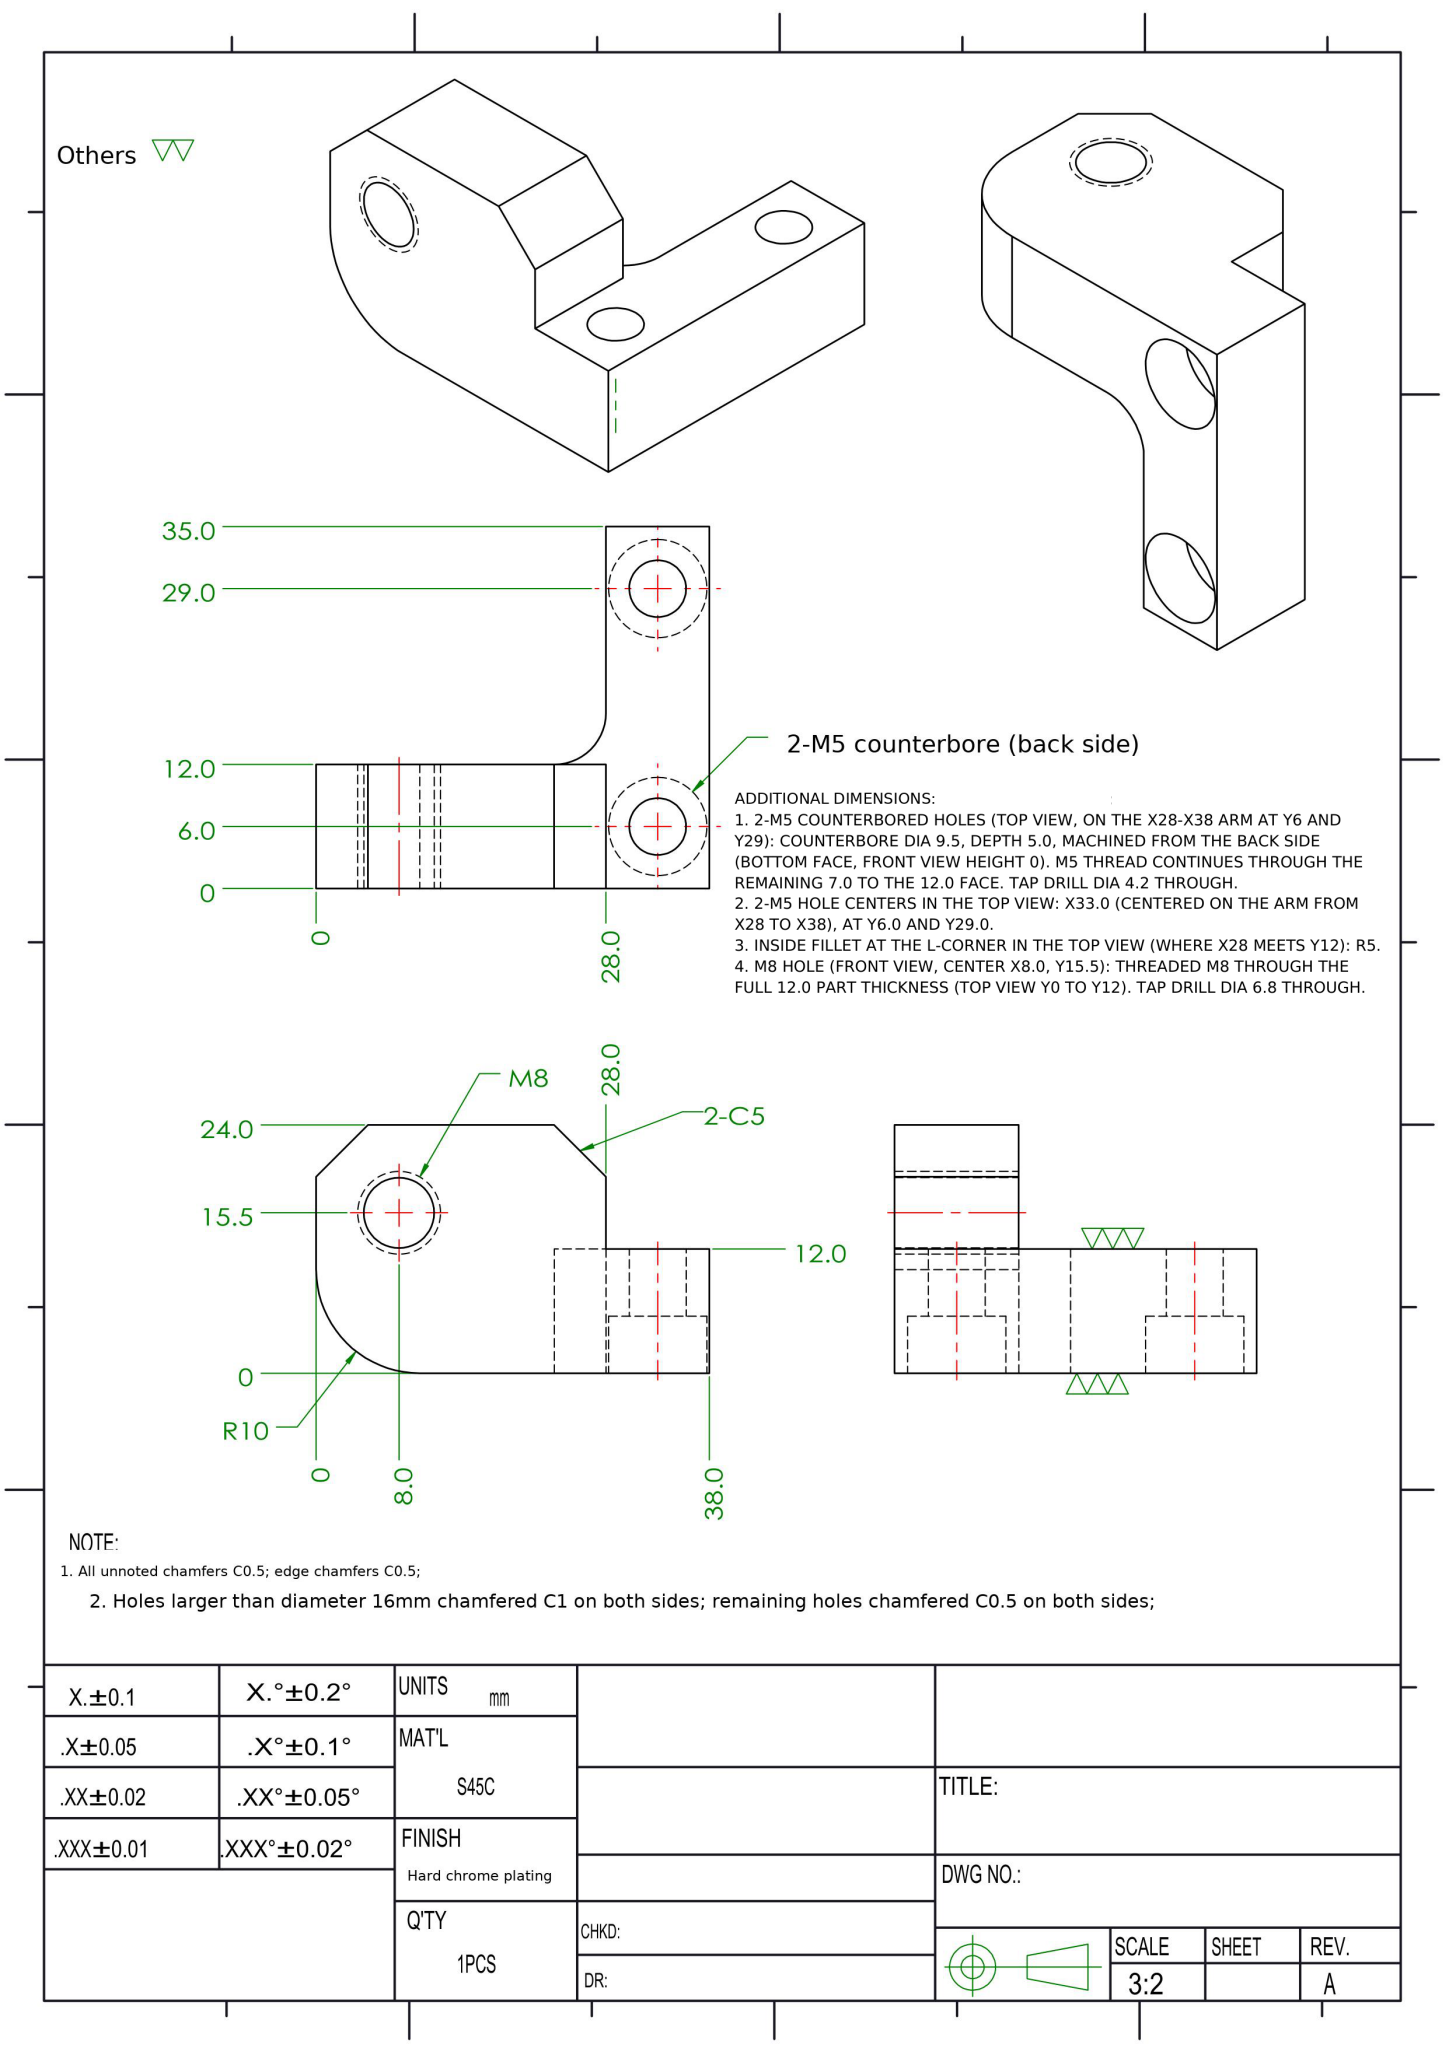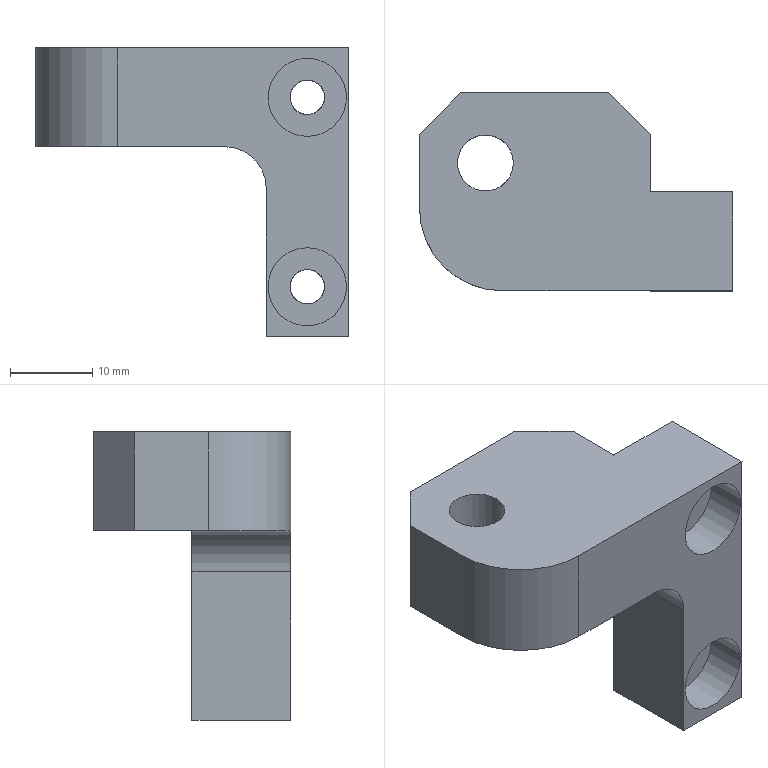Part | NX | mm | Stepped Dual-Bore Right-Angle Bracket 38mm | 1 solid | 29 faces | box 38 x 24 x 35.01 mm | volume 10389 mm3 | plane 16 | cylinder 9 | spline 4 | commonest cylinder face diameters 4.2 x2 9.5 x2 5 x2 10 x1 20 x1 6.8 x1